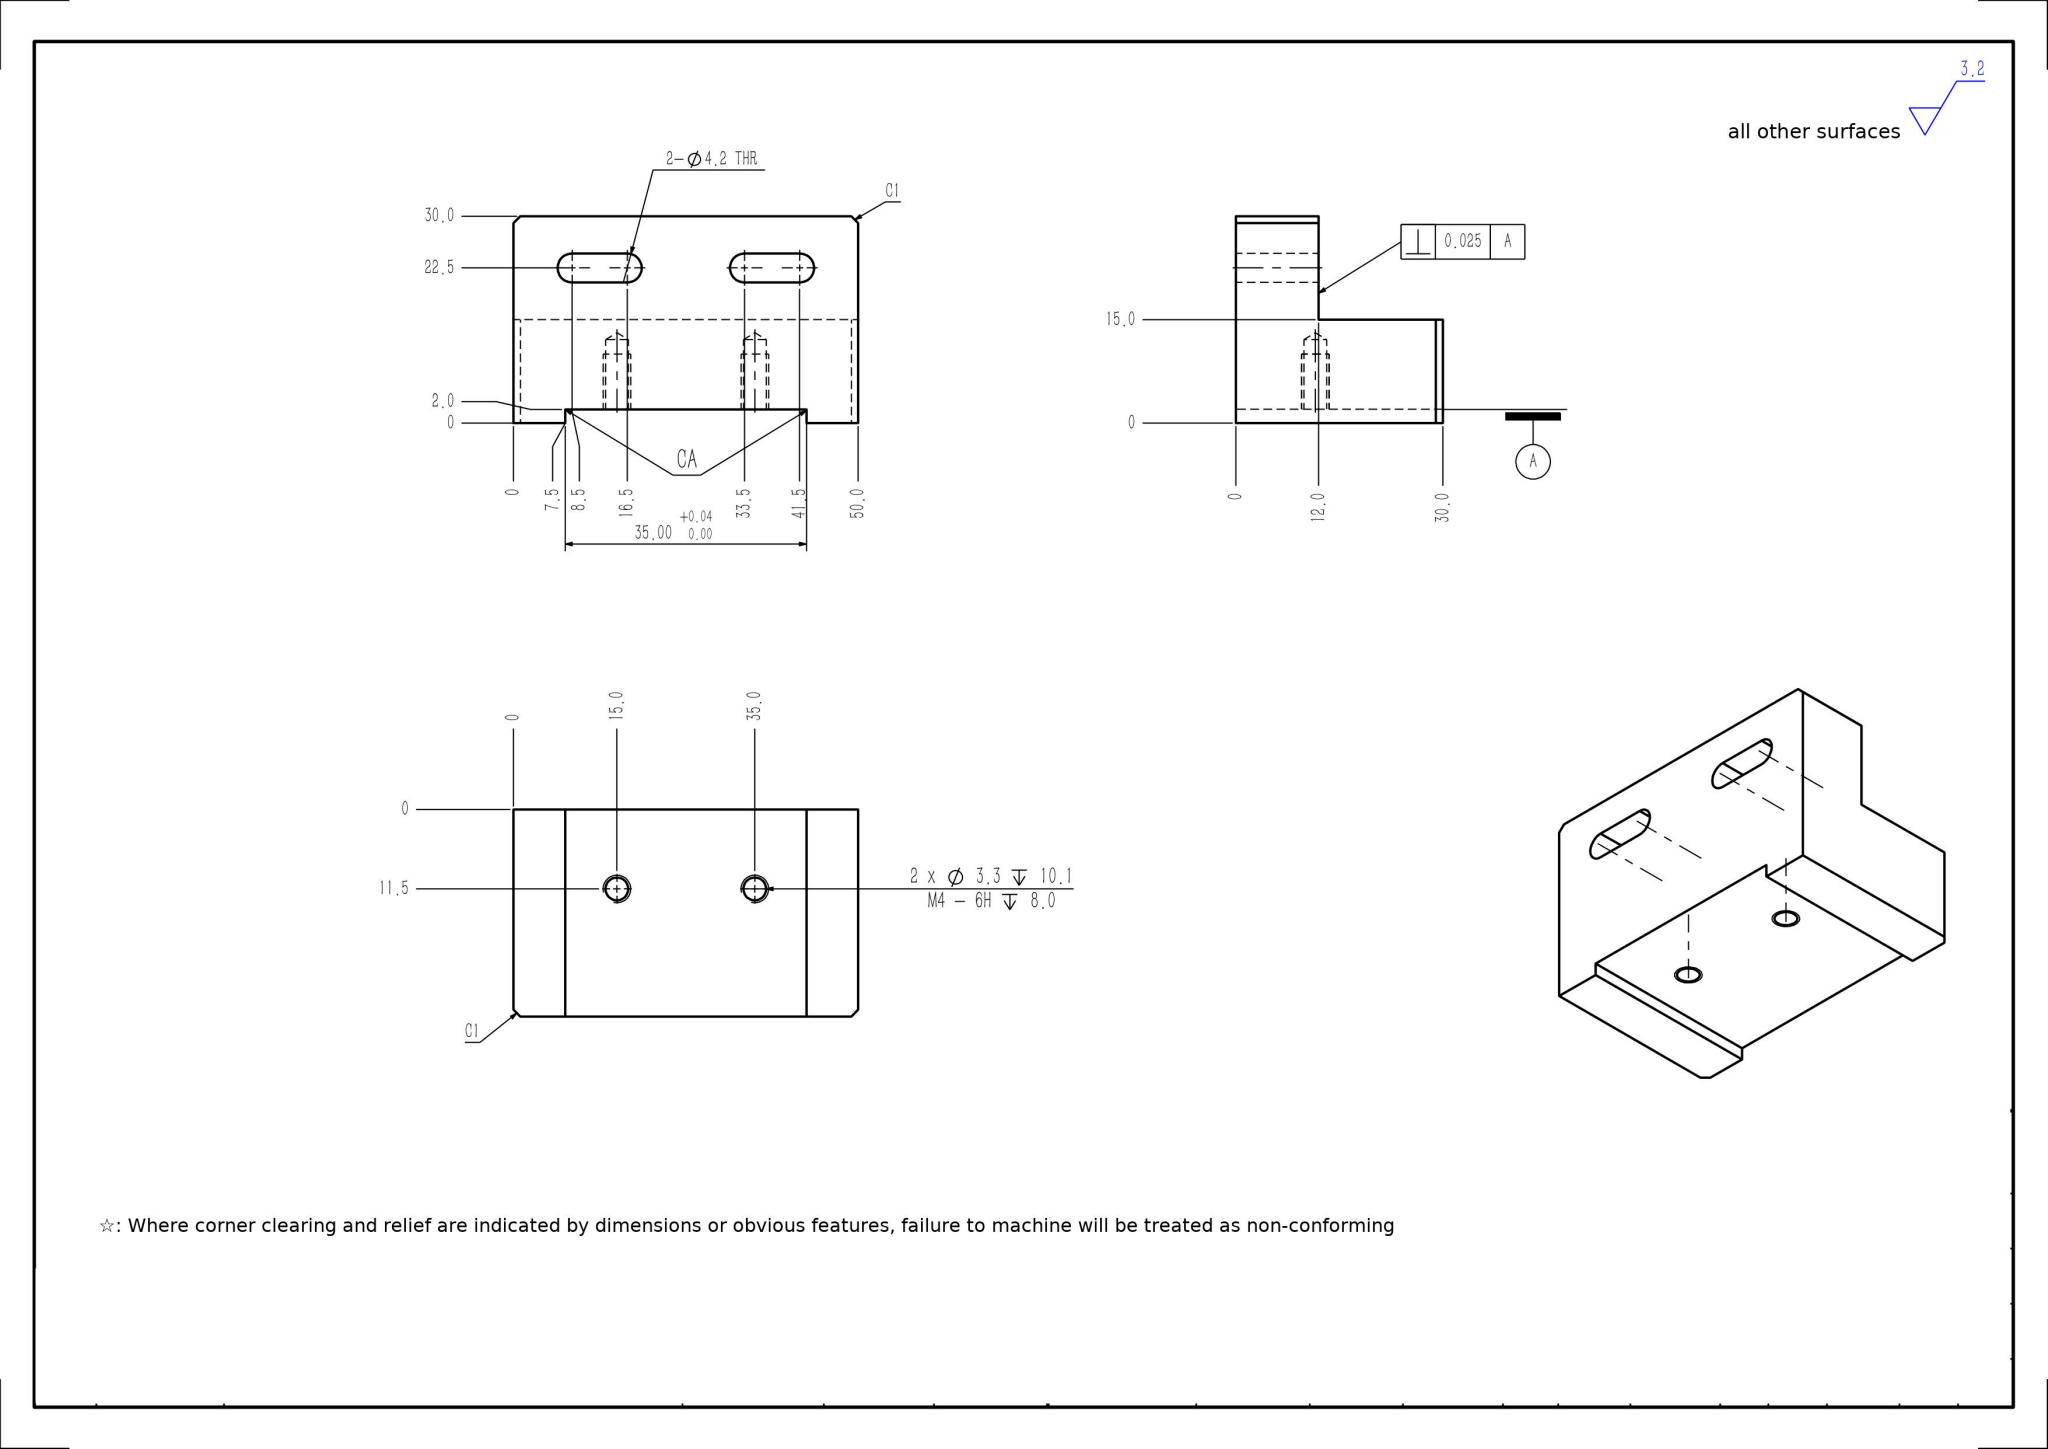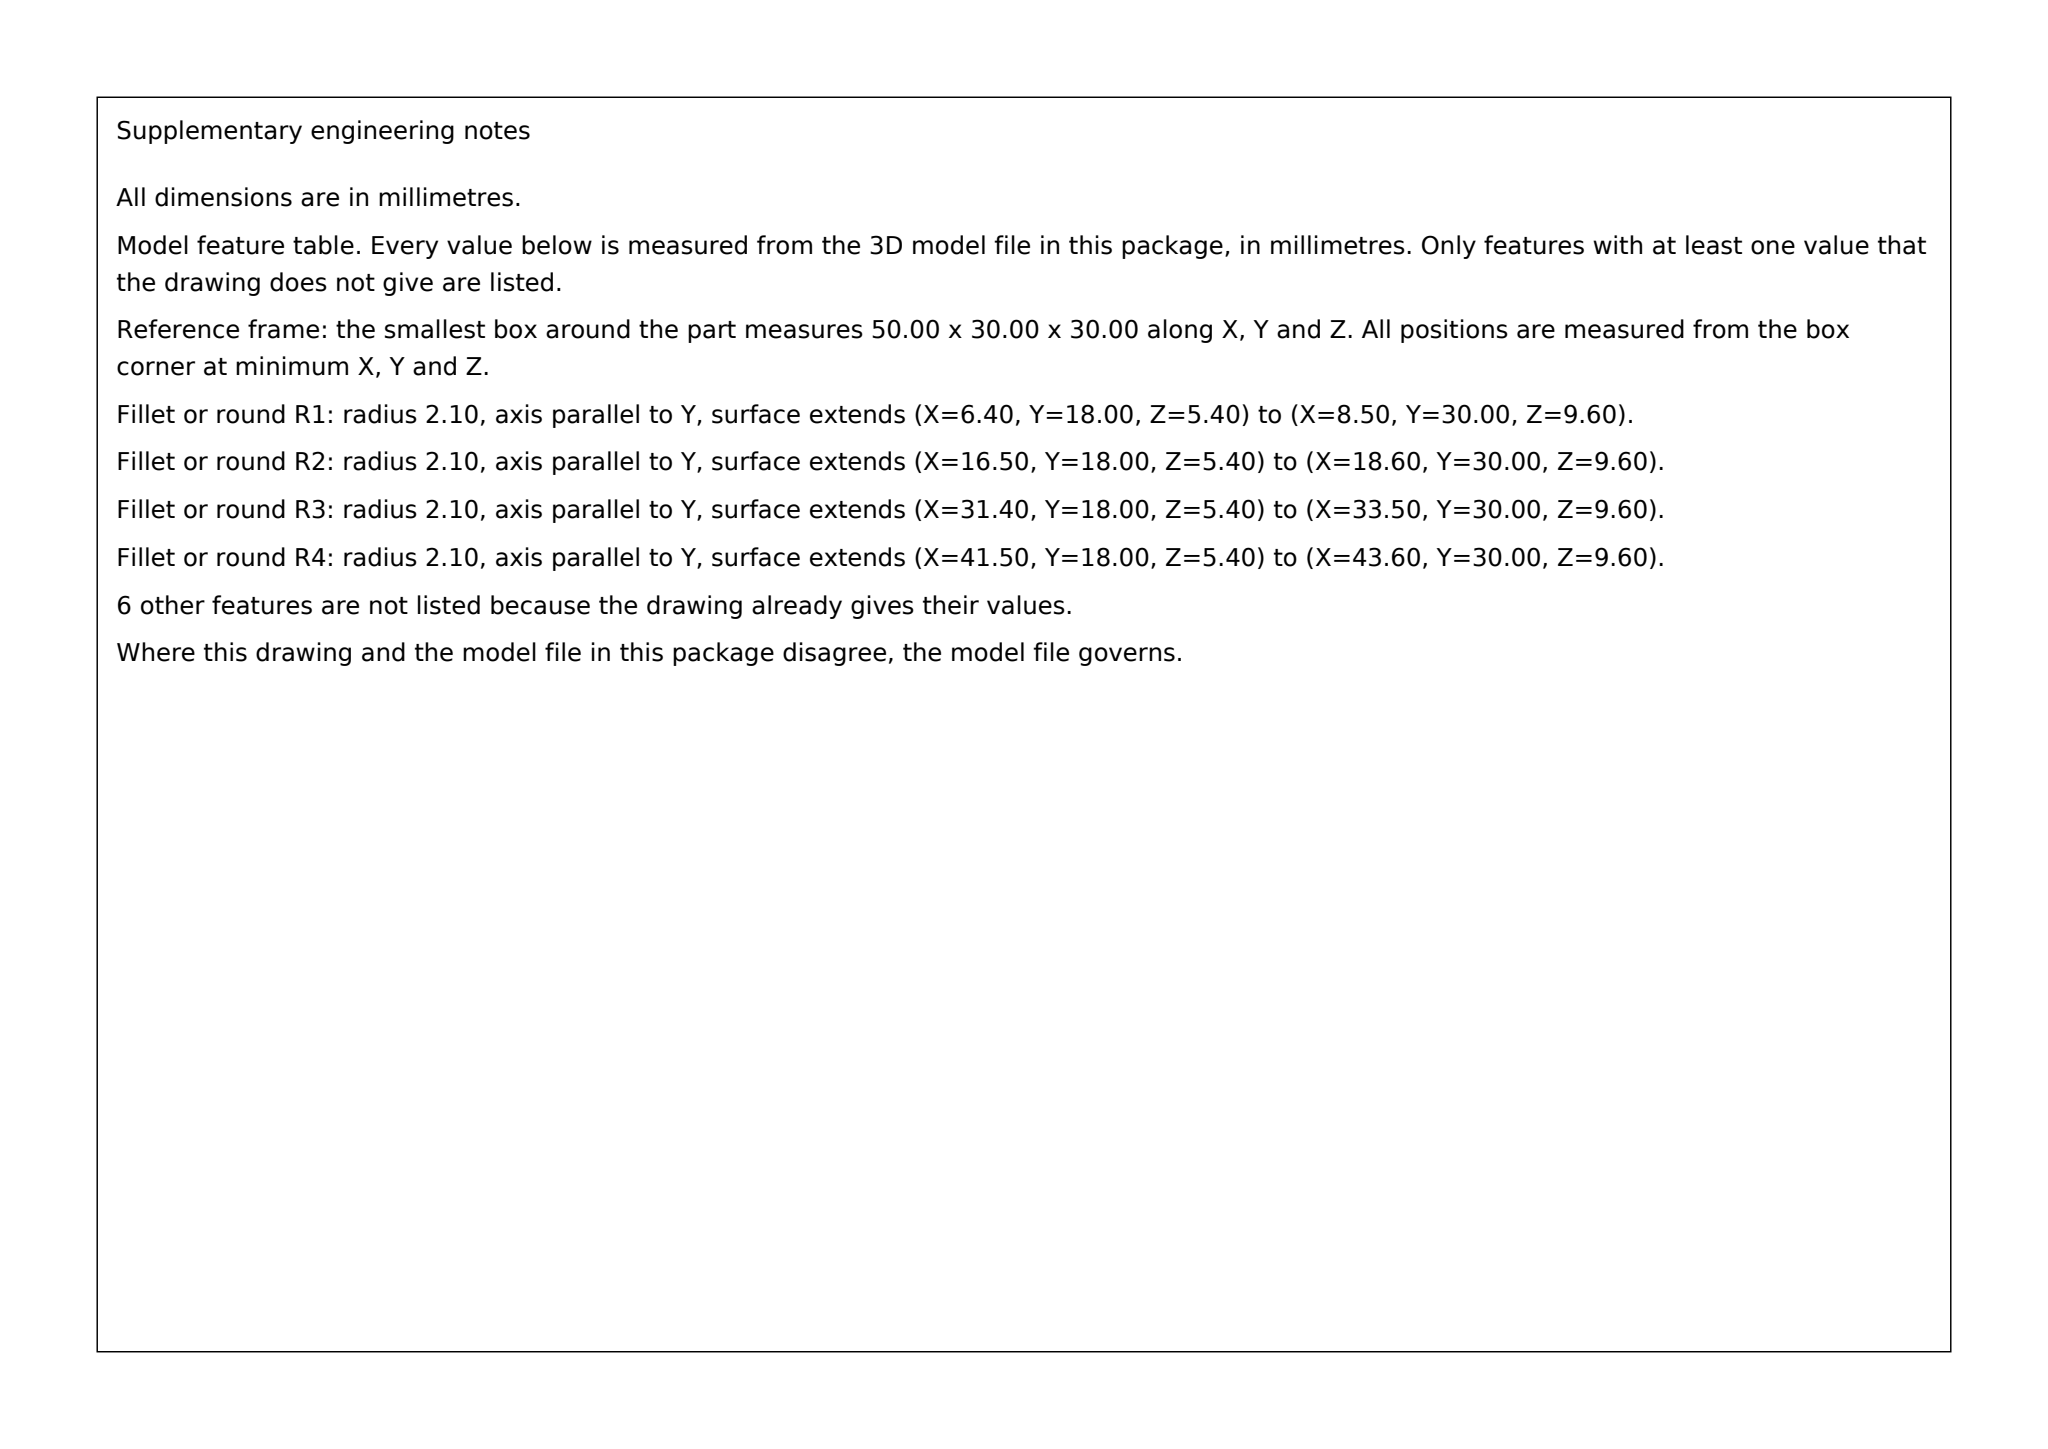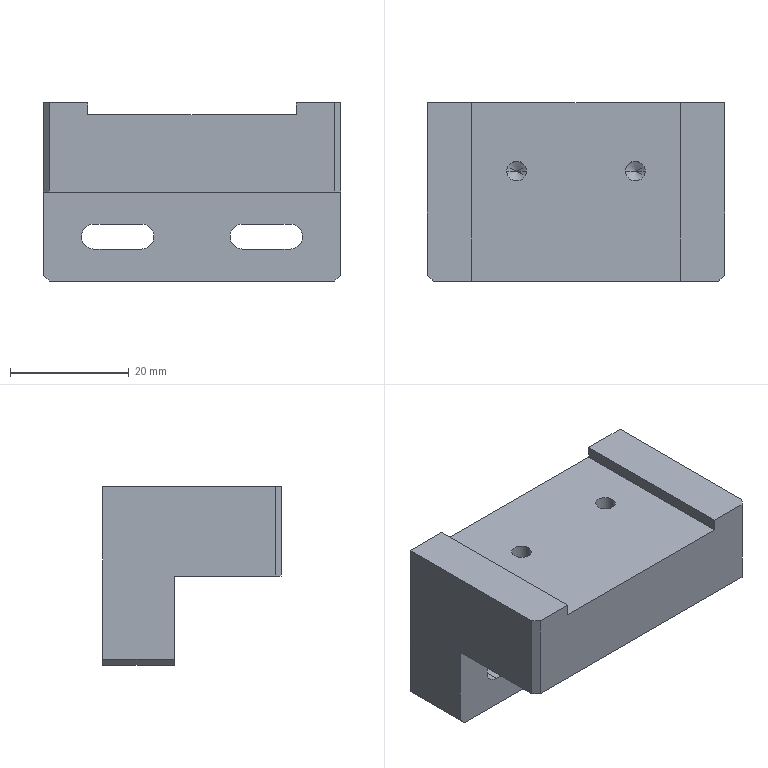Part | SolidWorks | mm | 1 solid | 32 faces | box 50 x 30 x 30 mm | volume 28056 mm3 | plane 20 | cylinder 8 | cone 4 | commonest cylinder face diameters 3.3 x4 4.2 x4
build123d program:
from build123d import *

# Parameters (mm, degrees)
SKETCH1_W                  = 50
SKETCH1_H                  = 30
BOSS_EXTRUDE1_DEPTH        = 15
SKETCH23_W                 = 60
SKETCH23_H                 = 18
CUT_EXTRUDE11_DEPTH        = 15
SKETCH16_W                 = 35
SKETCH16_H                 = 30
CUT_EXTRUDE8_DEPTH         = 2
M4_TAPPED_HOLE1_D          = 3.3
M4_TAPPED_HOLE1_DEPTH      = 10.1
M4_TAPPED_HOLE1_TIP        = 0.9914
F_4_2_4_2_DIAMETER_HOLE1_D = 4.2
CUT_EXTRUDE12_DEPTH        = 42.833
CHAMFER4_SIZE              = 1


with BuildPart() as part:
    # Sketch1 → Boss-Extrude1 (new, symmetric)
    with BuildSketch(Plane(origin=(0, 0, 0), x_dir=(1, 0, 0), z_dir=(0, 1, 0))):
        Rectangle(SKETCH1_W, SKETCH1_H)
    extrude(amount=BOSS_EXTRUDE1_DEPTH, both=True)

    # Sketch23 → Cut-Extrude11 (cut)
    with BuildSketch(Plane(origin=(0, 0, -15), x_dir=(-1, 0, 0), z_dir=(0, 0, -1))):
        with Locations((0, -6)):
            Rectangle(SKETCH23_W, SKETCH23_H)
    extrude(amount=-CUT_EXTRUDE11_DEPTH, mode=Mode.SUBTRACT)

    # Sketch16 → Cut-Extrude8 (cut)
    with BuildSketch(Plane.XY.offset(15)):
        Rectangle(SKETCH16_W, SKETCH16_H)
    extrude(amount=-CUT_EXTRUDE8_DEPTH, mode=Mode.SUBTRACT)

    # M4 Tapped Hole1
    with Locations(Plane.XY.offset(13)):
        with Locations((10, 3.5), (-10, 3.5)):
            Hole(M4_TAPPED_HOLE1_D / 2, depth=M4_TAPPED_HOLE1_DEPTH)
            with Locations((0, 0, -(M4_TAPPED_HOLE1_DEPTH + M4_TAPPED_HOLE1_TIP / 2))):  # 118° drill point
                Cone(0, M4_TAPPED_HOLE1_D / 2, M4_TAPPED_HOLE1_TIP, mode=Mode.SUBTRACT)

    # 4.2 _4.2_ Diameter Hole1 (through all)
    with Locations(Plane(origin=(0, 15, 0), x_dir=(1, 0, 0), z_dir=(0, 1, 0))):
        with Locations((-12.5, 7.5), (12.5, 7.5)):
            Hole(F_4_2_4_2_DIAMETER_HOLE1_D / 2)

    # Sketch28 → Cut-Extrude12 (cut, through all)
    with BuildSketch(Plane(origin=(0, 15, 0), x_dir=(1, 0, 0), z_dir=(0, 1, 0))):
        with BuildLine():
            Line((-16.5, 9.6), (-8.5, 9.6))
            ThreePointArc((-8.5, 9.6), (-6.4, 7.5), (-8.5, 5.4))
            Line((-8.5, 5.4), (-16.5, 5.4))
            ThreePointArc((-16.5, 5.4), (-18.6, 7.5), (-16.5, 9.6))
        make_face()
        with BuildLine():
            Line((8.5, 9.6), (16.5, 9.6))
            ThreePointArc((16.5, 9.6), (18.6, 7.5), (16.5, 5.4))
            Line((16.5, 5.4), (8.5, 5.4))
            ThreePointArc((8.5, 5.4), (6.4, 7.5), (8.5, 9.6))
        make_face()
    extrude(amount=-CUT_EXTRUDE12_DEPTH, mode=Mode.SUBTRACT)

    # Chamfer4
    chamfer4_edges = [part.edges().sort_by_distance(p)[0] for p in [
        (-25, -15, 7.5),
        (25, -15, 7.5),
        (-25, 9, -15),
        (25, 9, -15),
    ]]
    chamfer(chamfer4_edges, length=CHAMFER4_SIZE)


solid = part.part